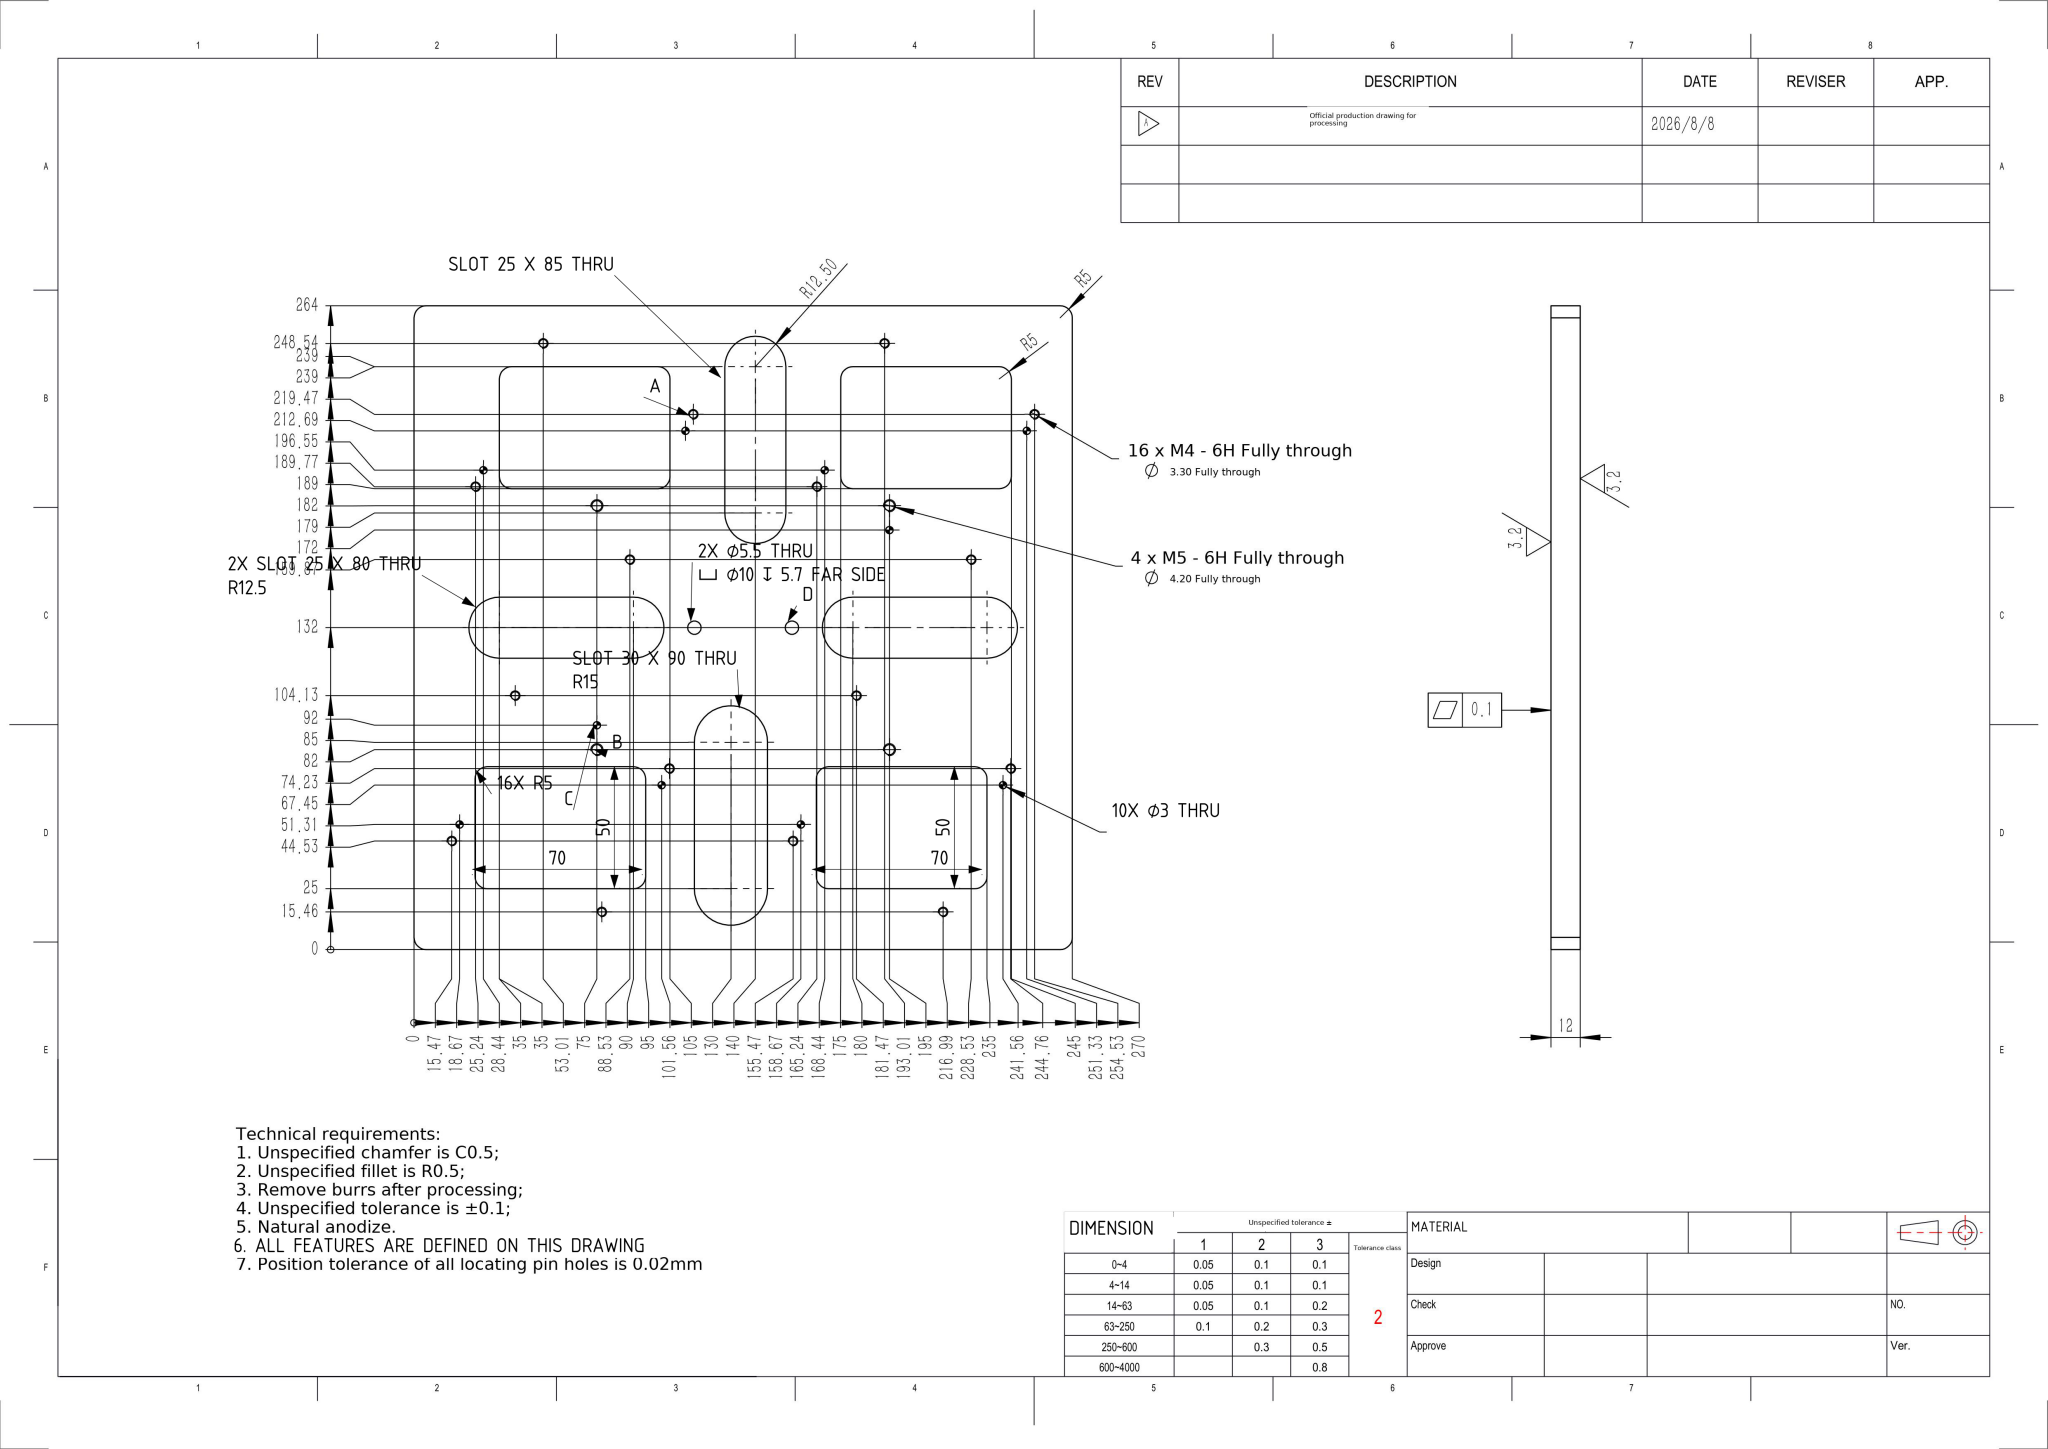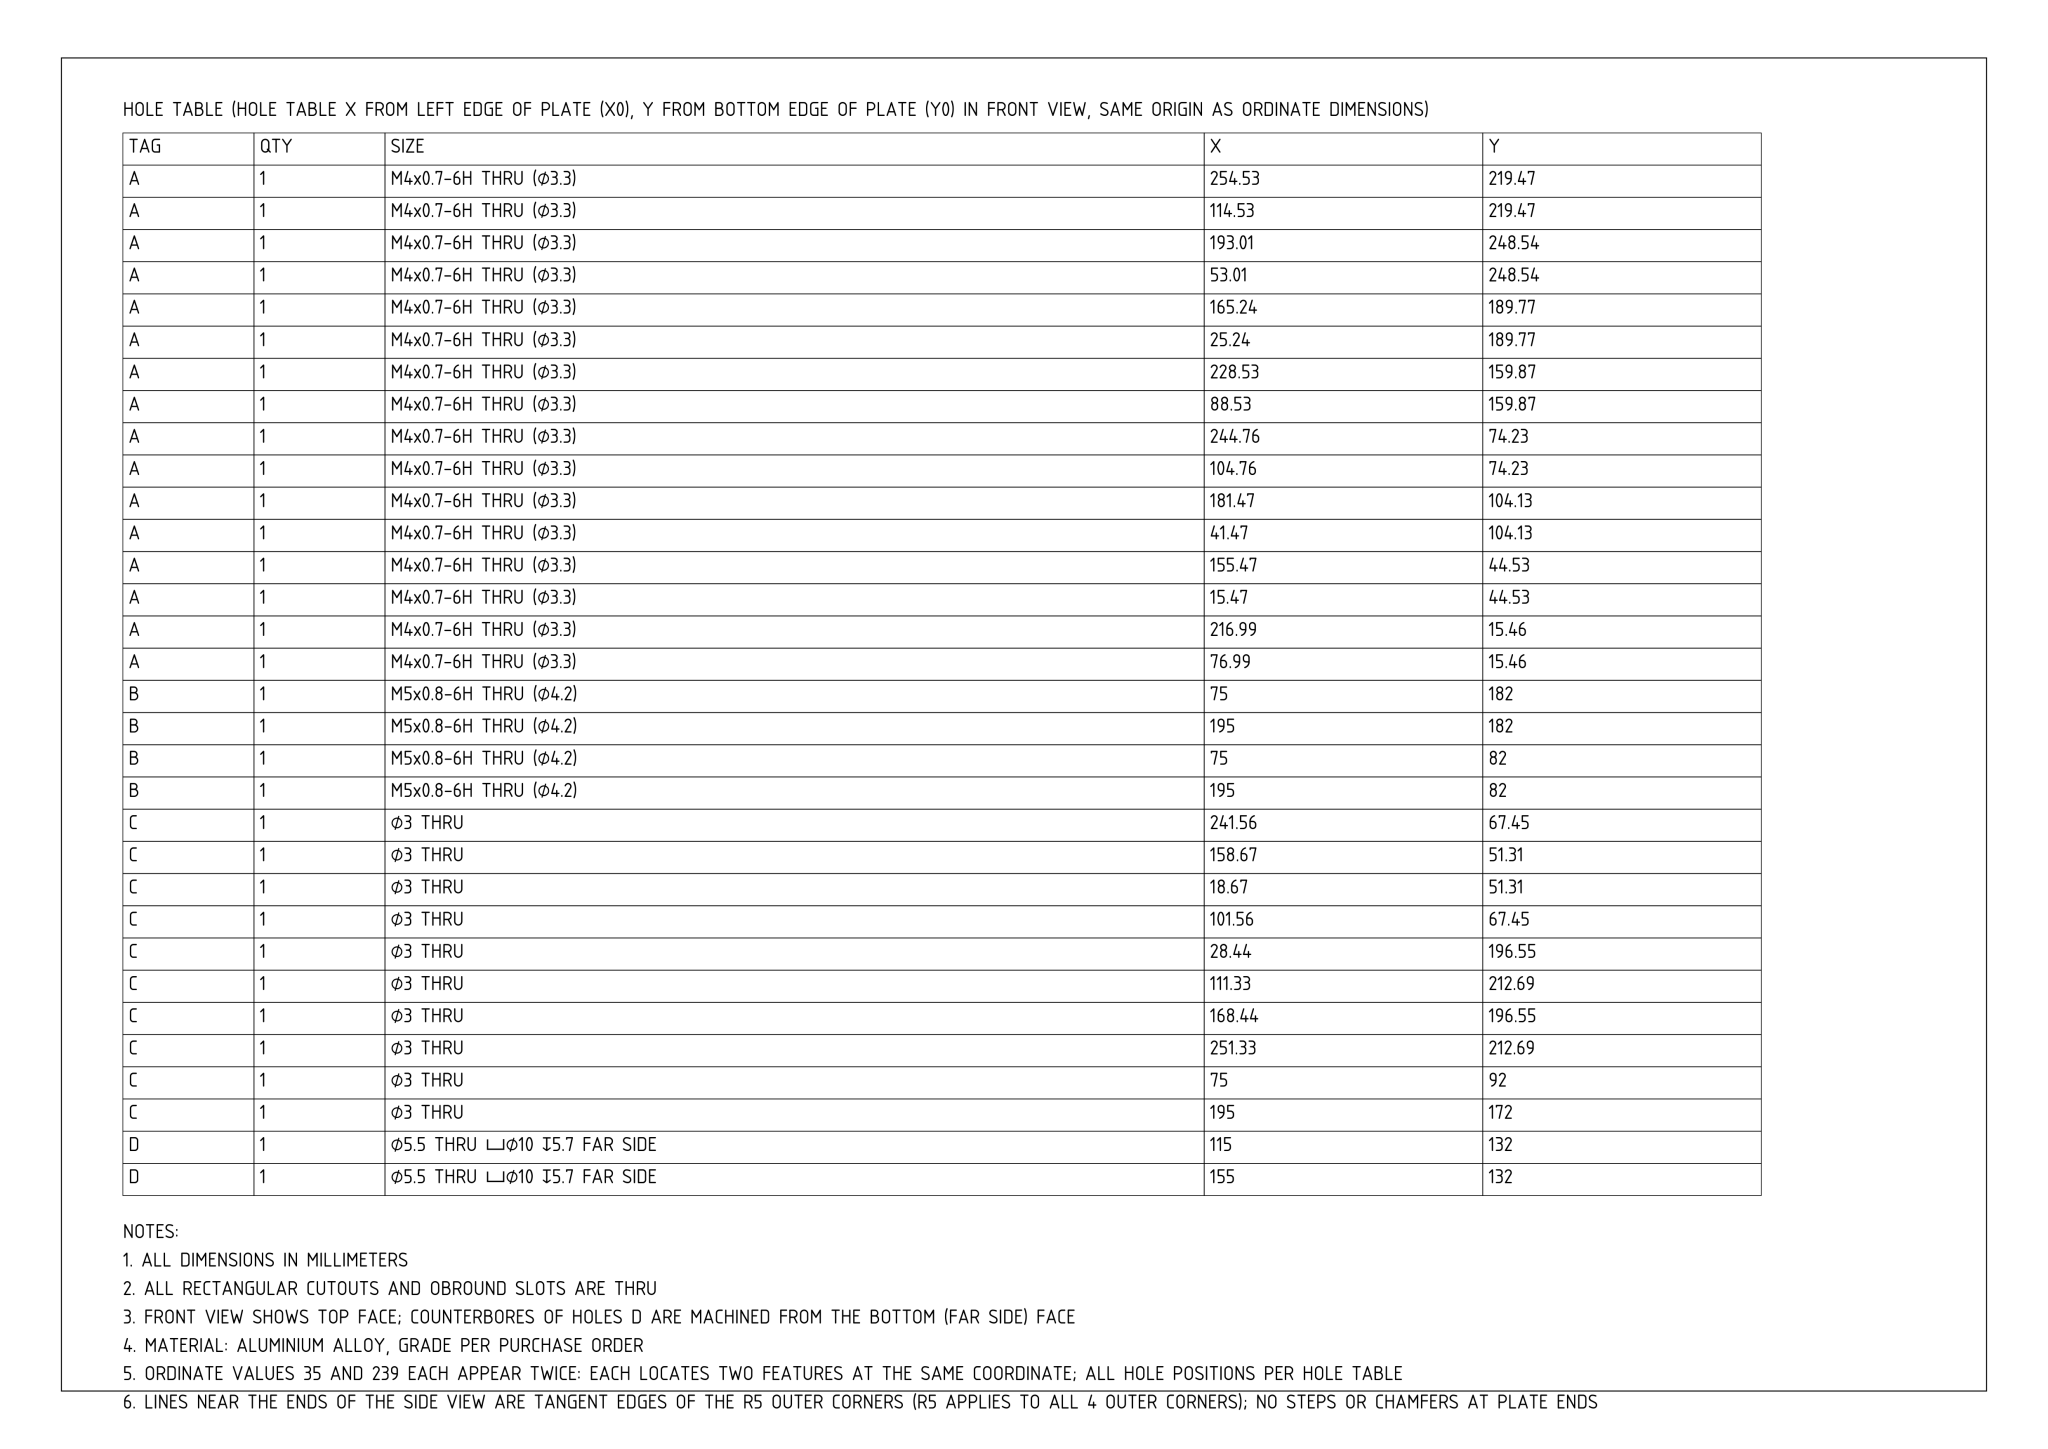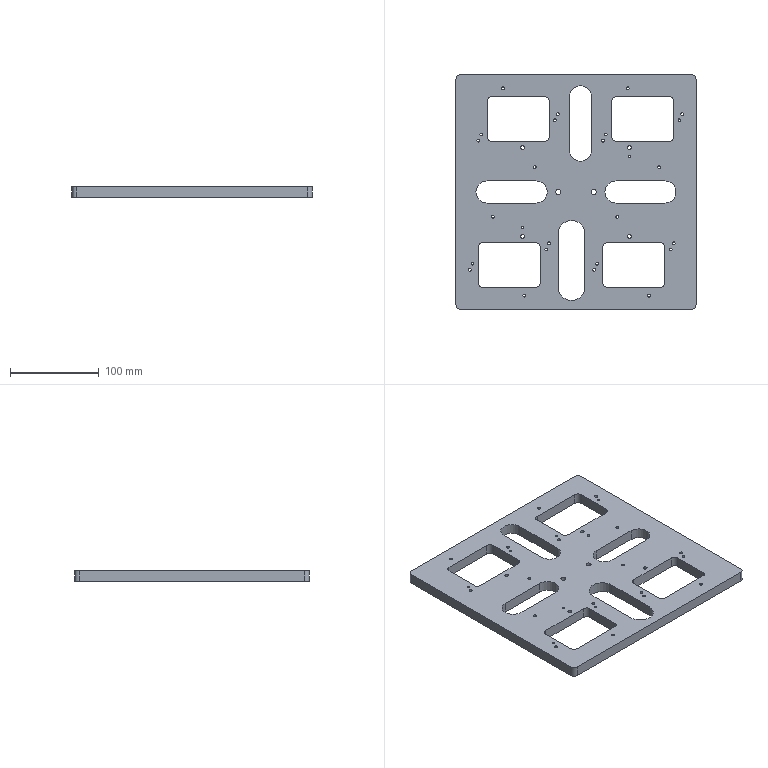Part | NX | mm | 1 solid | 130 faces | box 270 x 264 x 12 mm | volume 585029 mm3 | cylinder 98 | plane 32 | commonest cylinder face diameters 3.3 x32 10 x24 3 x20 25 x8 4.2 x8 5.5 x4 30 x2